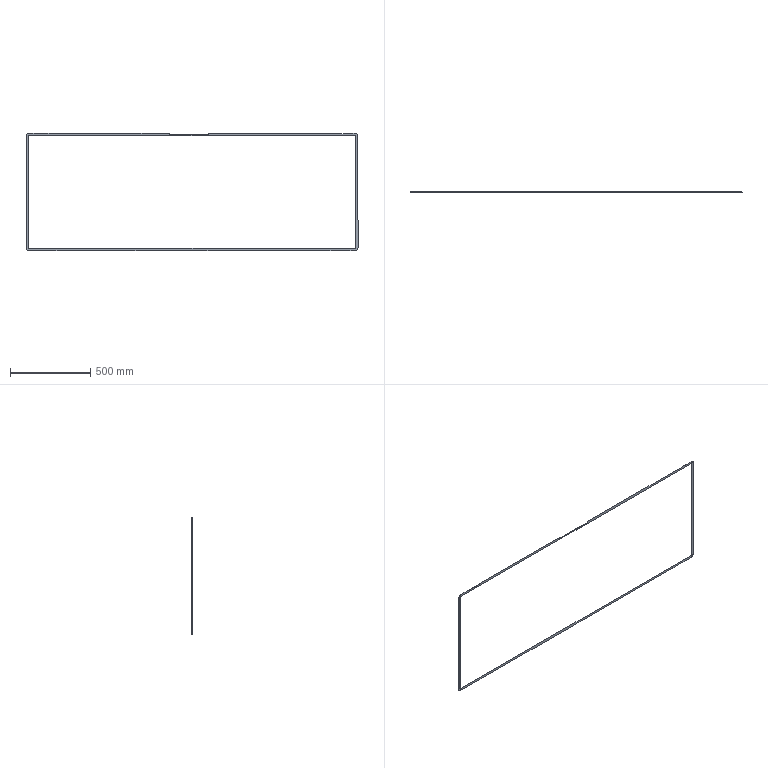Component | SolidWorks | FrontDoorAssembly-1_FrontDoorSealStrip-1 | 1 solid | 34 faces | volume 164879 mm3 | plane 25 | cylinder 5 | torus 4 | commonest cylinder face diameters 21.75 x5